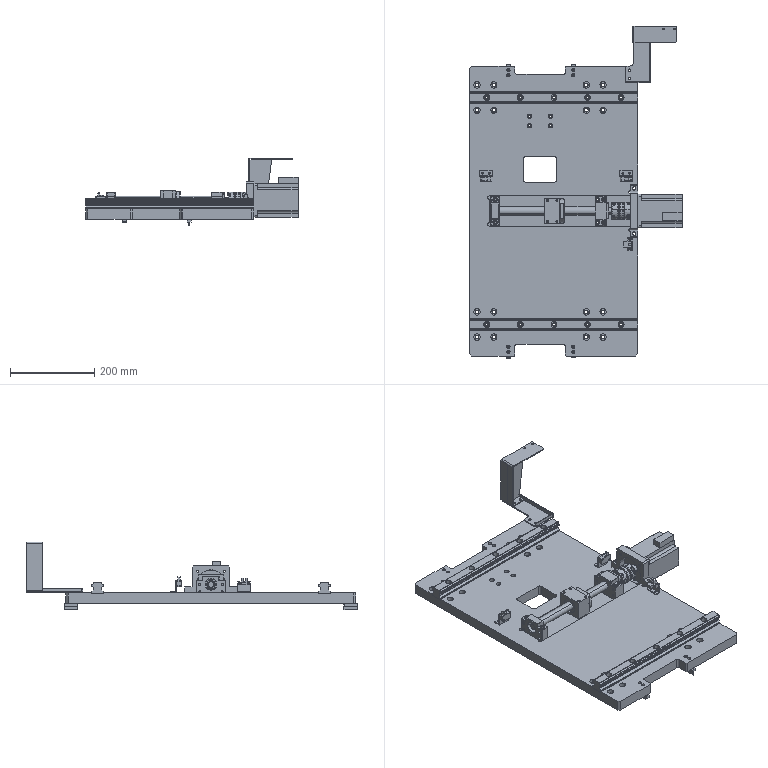Assembly | SolidWorks | mm | 27 component files | 28 solids | 1819 faces | box 505 x 789.7 x 161.7 mm | volume 7869612 mm3 | plane 909 | cylinder 651 | spline 127 | cone 126 | torus 6 | commonest cylinder face diameters 9 x52 5 x42 4 x40 15 x40 5.5 x40 6 x34 3.3 x32 4.2 x24
Bill of materials:
6G-DCSG-StopSwitchSeat | 2 |  | L-shaped angle bracket: a tall rectangular vertical plate joined at a right angle to a short horizontal foot. The vertical plate has four small holes near its upper portion and the foot has two larger holes.
6G-DCSG-ZeroPointSwitchSeat | 1 |  | L-shaped angle bracket: a wide rectangular vertical plate with a narrower horizontal foot. The vertical plate has two small holes near its top edge and the foot has two larger holes.
6G-HGR30-Y-Integrated | 2 |  | Long straight rail with a constant profile. Both sides have lengthwise grooves, and a row of evenly spaced counterbored holes runs along the top face.
6G-LimitSwitch | 2 |  | Small rectangular block with rounded corners and two through holes at diagonally opposite corners. On top there is a raised tab with a rounded end and a thin angled strip that slopes along the top face.
6G-OriginSwitch | 1 |  | Stepped rectangular block with two parallel upright prongs that form an open slot between them. Holes run both vertically and horizontally through the lower flange sections.
6G-TL06.01.02-XAxisMovingBasePlate | 1 |  | Large flat rectangular plate with many holes. It has a rectangular through-cutout, rectangular notches at both short ends, a shallow notch along one long edge, and shallow grooves or steps across the top face.
6G-TL06.01.05-DragChainFixingPlate | 1 |  | Formed thin-walled bracket: a tapered vertical web with a horizontal top flange and a horizontal bottom flange, joined by rounded bends. The top flange has two holes and the bottom flange has about three or four.
6G-TL06-StopBlock | 2 |  | Rectangular bar block with two round holes through its top face and one chamfered lower edge at one end.
6G-TL06-X-AxisCableCarrierBracket-A | 1 | AISI 304 | Thin flat plate with a stepped outline: a wide end and a narrower main body joined by a concave fillet. A narrow lip is turned down along one long edge. There are six round holes, and some corners are chamfered.
6G-TL06-X-AxisOrigin | 2 |  | Long bar with a T-shaped cross-section: a wide top flange over a narrower tongue underneath. Two round holes go into the top face.
6G-BF15SupportSide | 1 |  | Rectangular housing block with a raised centre section and a large central through bore. Four smaller holes go through the front face, two counterbored holes go down through the side shoulders, and the edges are chamfered.
6G-BK15FixedSide | 1 |  | Rectangular housing block with a raised centre section and a protruding flange boss on one face. A stepped central bore passes through it. There are four small holes around the bore on the boss, four through holes in the front face, and four counterbored vertical holes in the side shoulders.
6G-CPDW40-12-19 | 1 |  | Cylindrical body with a coaxial through-bore, made of two end hubs and a center ring. Thin disc-like layers sit in the gaps between them. Each hub has a slit and tangential cross holes with counterbores. The shape matches a clamp-style flexible shaft coupling.
6G-M4 | 4 |  | Headed fastener-like part: a cylindrical head with a hexagonal socket recess and a plain cylindrical shank with a chamfered tip. The shape matches a socket head cap screw.
6G-SGM7J-08A(750W) | 1 |  | Prismatic housing with a square front flange, four corner through-holes and a cylindrical output shaft sticking out from a round pilot boss. It has longitudinal grooves along the sides and a rectangular block on top. The shape matches a simplified motor (e.g., stepper or servo) envelope.
6G-TL06.01.03-X-AxisMotorMountingPlate | 1 |  | Flat rectangular plate with chamfered corners and a large central circular through-opening. Four small holes sit on a square pattern around the opening. Two side tabs at the base each have a through-hole perpendicular to the plate. The shape matches a mounting bracket or flange adapter plate.
6G-TL06.01.04-X-AxisFlangeMountingBlock | 1 |  | Rectangular block with a large circular through-bore along one axis. Four small holes surround the bore on the bore face, and four holes are in the top face. The shape matches a housing or nut block.
6G-TL06-Y-AxisFlange | 1 |  | Flanged cylindrical bushing with a central through-bore. The flange is round with two parallel flats and six through-holes. The shape matches a flanged lead-screw nut or flanged bushing.
6G-TL06-Y-AxisScrew | 1 |  | Long, slender stepped round shaft. A long main diameter steps down at one end into two progressively smaller journals. The other end has a short, slightly reduced section.
Mates:
1. concentric | 6G-DCSG-StopSwitchSeat-1 face at (-150.85, 83.8, 27) dir (0, 1, 0) r 1.25 | 6G-LimitSwitch-1 face at (-150.85, 71, 27) dir (0, 1, 0) r 1.75
2. coincident | 6G-DCSG-StopSwitchSeat-1 face at (-177, 83.8, 30) dir (0, 0, 1) | 6G-LimitSwitch-1 face at (-149.85, 81, 30) dir (0, 0, 1)
3. coincident | 6G-DCSG-StopSwitchSeat-1 face at (-177, 81, 30) dir (0, -1, 0) | 6G-LimitSwitch-1 face at (-149.85, 81, 16) dir (0, 1, 0)
4. concentric | 6G-DCSG-StopSwitchSeat-2 face at (160.85, 83.8, 27) dir (0, 1, 0) r 1.25 | 6G-LimitSwitch-2 face at (160.85, 81, 27) dir (0, -1, 0) r 1.75
5. coincident | 6G-DCSG-StopSwitchSeat-2 face at (157, 83.8, 30) dir (0, 0, 1) | 6G-LimitSwitch-2 face at (159.85, 71, 30) dir (0, 0, 1)
6. coincident | 6G-DCSG-StopSwitchSeat-2 face at (157, 81, 30) dir (0, -1, 0) | 6G-LimitSwitch-2 face at (159.85, 81, 16) dir (0, 1, 0)
7. concentric | 6G-DCSG-ZeroPointSwitchSeat-1 face at (184.472, -88.5, 22.3) dir (-1, 0, 0) r 1.25 | 6G-OriginSwitch-1 face at (187.872, -88.5, 22.3) dir (-1, 0, 0) r 1.5
8. parallel | 6G-DCSG-ZeroPointSwitchSeat-1 face at (187.272, -94, 26) dir (0, 0, 1) | 6G-OriginSwitch-1 face at (187.872, -95.044, 25.8) dir (0, 0, 1)
9. coincident | 6G-TL06.01.02-XAxisMovingBasePlate-1 face at (0, 0, -25) dir (0, 0, -1) | 6G-TL06-StopBlock-2 face at (-103.5, 349.7, -25) dir (0, 0, 1)
10. coincident | 6G-TL06.01.02-XAxisMovingBasePlate-1 face at (0, 0, -25) dir (0, 0, -1) | 6G-TL06-X-AxisOrigin-1 face at (46, 333, -25) dir (0, 0, 1)
11. coincident | 6G-TL06.01.02-XAxisMovingBasePlate-1 face at (0, 0, -25) dir (0, 0, -1) | 6G-TL06-StopBlock-2 face at (-103.5, 349.7, -25) dir (0, 0, 1)
12. coincident | 6G-TL06.01.02-XAxisMovingBasePlate-1 face at (0, 0, -25) dir (0, 0, -1) | 6G-TL06-X-AxisOrigin-1 face at (46, 333, -25) dir (0, 0, 1)
13. coincident | 6G-DCSG-StopSwitchSeat-1 face at (-177, 96, 0) dir (0, 0, -1) | 6G-TL06.01.02-XAxisMovingBasePlate-1 face at (0, 0, 0) dir (0, 0, 1)
14. coincident | 6G-DCSG-StopSwitchSeat-2 face at (157, 96, 0) dir (0, 0, -1) | 6G-TL06.01.02-XAxisMovingBasePlate-1 face at (0, 0, 0) dir (0, 0, 1)
15. coincident | 6G-DCSG-ZeroPointSwitchSeat-1 face at (175.272, -94, 0) dir (0, 0, -1) | 6G-TL06.01.02-XAxisMovingBasePlate-1 face at (0, 0, 0) dir (0, 0, 1)
16. coincident | 6G-TL06.01.02-XAxisMovingBasePlate-1 face at (0, 0, -2.5) dir (0, 0, 1) | 6G-HGR30-Y-Integrated-2 face at (-140, 262.25, -2.5) dir (0, 0, -1)
17. width | 6G-HGR30-Y-Integrated-2 face at (-140, 284, 2.61) dir (0, 1, 0) | 6G-HGR30-Y-Integrated-2 face at (-140, 256, -1) dir (0, -1, 0) | 6G-TL06.01.02-XAxisMovingBasePlate-1 face at (-200, 284, -2.5) dir (0, -1, 0) | 6G-TL06.01.02-XAxisMovingBasePlate-1 face at (-200, 256, -2.5) dir (0, 1, 0)
18. coincident | 6G-TL06.01.02-XAxisMovingBasePlate-1 face at (0, 0, -2.5) dir (0, 0, 1) | 6G-HGR30-Y-Integrated-3 face at (-140, -277.75, -2.5) dir (0, 0, -1)
19. width | 6G-HGR30-Y-Integrated-3 face at (-140, -284, -1) dir (0, -1, 0) | 6G-HGR30-Y-Integrated-3 face at (-140, -256, 2.61) dir (0, 1, 0) | 6G-TL06.01.02-XAxisMovingBasePlate-1 face at (-200, -284, -2.5) dir (0, 1, 0) | 6G-TL06.01.02-XAxisMovingBasePlate-1 face at (-200, -256, -2.5) dir (0, -1, 0)
20. width | 6G-HGR30-Y-Integrated-3 face at (-200, -220, -2.5) dir (-1, 0, 0) | 6G-HGR30-Y-Integrated-3 face at (200, -220, -2.5) dir (1, 0, 0) | 6G-TL06.01.02-XAxisMovingBasePlate-1 face at (200, -345, -25) dir (1, 0, 0) | 6G-TL06.01.02-XAxisMovingBasePlate-1 face at (-200, -345, -25) dir (-1, 0, 0)
21. width | 6G-HGR30-Y-Integrated-2 face at (-200, 320, -2.5) dir (-1, 0, 0) | 6G-HGR30-Y-Integrated-2 face at (200, 320, -2.5) dir (1, 0, 0) | 6G-TL06.01.02-XAxisMovingBasePlate-1 face at (200, -345, -25) dir (1, 0, 0) | 6G-TL06.01.02-XAxisMovingBasePlate-1 face at (-200, -345, -25) dir (-1, 0, 0)
22. coincident | 6G-TL06.01.02-XAxisMovingBasePlate-1 face at (0, 0, 0) dir (0, 0, 1) | 6G-TL06-Y-AxisMotorAssembly-2/6G-TL06.01.03-X-AxisMotorMountingPlate-1 face at (222.672, 45, 0) dir (0, 0, -1)
23. width | 6G-TL06-Y-AxisMotorAssembly-2/6G-TL06.01.03-X-AxisMotorMountingPlate-1 face at (222.672, 62, 0) dir (0, 1, 0) | 6G-TL06-Y-AxisMotorAssembly-2/6G-TL06.01.03-X-AxisMotorMountingPlate-1 face at (222.672, -62, 0) dir (0, -1, 0) | 6G-TL06.01.02-XAxisMovingBasePlate-1 face at (200, -45, -25) dir (0, 1, 0) | 6G-TL06.01.02-XAxisMovingBasePlate-1 face at (200, 45, -25) dir (0, -1, 0)
24. coincident | 6G-TL06.01.02-XAxisMovingBasePlate-1 face at (182, 45, -25) dir (1, 0, 0) | 6G-TL06-Y-AxisMotorAssembly-2/6G-TL06.01.03-X-AxisMotorMountingPlate-1 face at (182, 0, 21.75) dir (-1, 0, 0)
25. concentric | 6G-TL06.01.02-XAxisMovingBasePlate-1 face at (-108.5, 323, 0) dir (0, 0, 1) r 2.25 | 6G-TL06-StopBlock-2 face at (-108.5, 323, -25) dir (0, 0, 1) r 1.65
26. concentric | 6G-TL06.01.02-XAxisMovingBasePlate-1 face at (-108.5, 335, 0) dir (0, 0, 1) r 2.25 | 6G-TL06-StopBlock-2 face at (-108.5, 335, -25) dir (0, 0, 1) r 1.65
27. concentric | 6G-TL06.01.02-XAxisMovingBasePlate-1 face at (-108.5, -323, 0) dir (0, 0, 1) r 2.25 | 6G-TL06-StopBlock-3 face at (-108.5, -323, -25) dir (0, 0, 1) r 1.65
28. concentric | 6G-TL06.01.02-XAxisMovingBasePlate-1 face at (-108.5, -335, 0) dir (0, 0, 1) r 2.25 | 6G-TL06-StopBlock-3 face at (-108.5, -335, -25) dir (0, 0, 1) r 1.65
29. coincident | 6G-TL06.01.02-XAxisMovingBasePlate-1 face at (0, 0, -25) dir (0, 0, -1) | 6G-TL06-StopBlock-3 face at (-113.5, -349.7, -25) dir (0, 0, 1)
30. concentric | 6G-TL06.01.02-XAxisMovingBasePlate-1 face at (46, 323, 0) dir (0, 0, 1) r 2.25 | 6G-TL06-X-AxisOrigin-1 face at (46, 323, -31.5) dir (0, 0, -1) r 1.65
31. concentric | 6G-TL06.01.02-XAxisMovingBasePlate-1 face at (46, 335, 0) dir (0, 0, 1) r 2.25 | 6G-TL06-X-AxisOrigin-1 face at (46, 335, -31.5) dir (0, 0, -1) r 1.65
32. concentric | 6G-DCSG-StopSwitchSeat-2 face at (164, 90, -7.2) dir (0, 0, 1) r 2.1 | 6G-TL06.01.02-XAxisMovingBasePlate-1 face at (164, 90, 0) dir (0, 0, 1) r 1.65
33. concentric | 6G-DCSG-StopSwitchSeat-2 face at (180, 90, -7.2) dir (0, 0, 1) r 2.1 | 6G-TL06.01.02-XAxisMovingBasePlate-1 face at (180, 90, 0) dir (0, 0, 1) r 1.65
34. concentric | 6G-DCSG-ZeroPointSwitchSeat-1 face at (180, -72, -27.2) dir (0, 0, 1) r 2.1 | 6G-TL06.01.02-XAxisMovingBasePlate-1 face at (180, -72, 0) dir (0, 0, 1) r 1.65
35. concentric | 6G-DCSG-ZeroPointSwitchSeat-1 face at (180, -86, -27.2) dir (0, 0, 1) r 2.1 | 6G-TL06.01.02-XAxisMovingBasePlate-1 face at (180, -86, 0) dir (0, 0, 1) r 1.65
36. concentric | 6G-DCSG-StopSwitchSeat-1 face at (-170, 90, -7.2) dir (0, 0, 1) r 2.1 | 6G-TL06.01.02-XAxisMovingBasePlate-1 face at (-170, 90, 0) dir (0, 0, 1) r 1.65
37. concentric | 6G-DCSG-StopSwitchSeat-1 face at (-154, 90, -7.2) dir (0, 0, 1) r 2.1 | 6G-TL06.01.02-XAxisMovingBasePlate-1 face at (-154, 90, 0) dir (0, 0, 1) r 1.65
38. coincident | 6G-TL06.01.02-XAxisMovingBasePlate-1 face at (0, 0, 0) dir (0, 0, 1) | 6G-TL06-X-AxisCableCarrierBracket-A-1 face at (180, 355, 0) dir (0, 0, -1)
39. concentric | 6G-TL06.01.02-XAxisMovingBasePlate-1 face at (180, 315, 0) dir (0, 0, 1) r 2.5 | 6G-TL06-X-AxisCableCarrierBracket-A-1 face at (180, 315, 0) dir (0, 0, 1) r 3.1
40. concentric | 6G-TL06.01.02-XAxisMovingBasePlate-1 face at (180, 335, 0) dir (0, 0, 1) r 2.5 | 6G-TL06-X-AxisCableCarrierBracket-A-1 face at (180, 335, 0) dir (0, 0, 1) r 3.1
41. coincident | 6G-TL06.01.05-DragChainFixingPlate-1 face at (207.375, 411.5, 2.5) dir (0, 0, -1) | 6G-TL06-X-AxisCableCarrierBracket-A-1 face at (180, 355, 2.5) dir (0, 0, 1)
42. coincident | 6G-TL06.01.05-DragChainFixingPlate-1 face at (187.25, 440, 2.5) dir (0, 1, 0) | 6G-TL06-X-AxisCableCarrierBracket-A-1 edge at (227, 440, 0) dir (-1, 0, 0)
43. coincident | 6G-TL06.01.05-DragChainFixingPlate-1 face at (227.5, 440, 2.5) dir (1, 0, 0) | 6G-TL06-X-AxisCableCarrierBracket-A-1 face at (227.5, 305, 2.5) dir (-1, 0, 0)
44. coincident | 6G-DCSG-ZeroPointSwitchSeat-1 face at (184.472, -94, 30) dir (-1, 0, 0) | 6G-OriginSwitch-1 face at (184.472, -92.25, 15.8) dir (1, 0, 0)
45. concentric | 6G-TL06.01.02-XAxisMovingBasePlate-1 face at (46, -323, 0) dir (0, 0, 1) r 4 | 6G-TL06-X-AxisOrigin-2 face at (46, -323, -31.5) dir (0, 0, -1) r 1.65
46. concentric | 6G-TL06.01.02-XAxisMovingBasePlate-1 face at (46, -335, 0) dir (0, 0, 1) r 4 | 6G-TL06-X-AxisOrigin-2 face at (46, -335, -31.5) dir (0, 0, -1) r 1.65
47. coincident | 6G-TL06.01.02-XAxisMovingBasePlate-1 face at (0, 0, -25) dir (0, 0, -1) | 6G-TL06-X-AxisOrigin-2 face at (46, -333, -25) dir (0, 0, 1)
48. concentric | 6G-TL06-Y-AxisScrew-1 face at (-1.75, 0, 84) dir (0, 0, 1) r 10 | 6G-BK15FixedSide-1 face at (-1.75, 0, 57) dir (0, 0, 1) r 7.5
49. coincident | 6G-TL06-Y-AxisScrew-1 face at (-1.75, 0, 84) dir (0, 0, -1) | 6G-BK15FixedSide-1 face at (-29.75, 0, 84) dir (0, 0, 1)
50. parallel | 6G-BK15FixedSide-1 face at (18.25, 20, 57) dir (1, 0, 0) | 6G-BF15SupportSide-1 face at (18.25, 19, 312) dir (1, 0, 0)
51. concentric | 6G-TL06-Y-AxisScrew-1 face at (-1.75, 0, 84) dir (0, 0, 1) r 10 | 6G-BF15SupportSide-1 face at (-1.75, 0, 312) dir (0, 0, 1) r 13
52. distance | 6G-BF15SupportSide-1 face at (-29.75, 0, 312) dir (0, 0, -1) | 6G-BK15FixedSide-1 face at (-29.75, 0, 84) dir (0, 0, 1)
53. concentric | 6G-TL06-Y-AxisScrew-1 face at (-1.75, 0, 24) dir (0, 0, 1) r 6 | 6G-TL06.01.03-X-AxisMotorMountingPlate-1 face at (-1.75, 0, -18) dir (0, 0, 1) r 35
54. parallel | 6G-BK15FixedSide-1 face at (18.25, 20, 57) dir (1, 0, 0) | 6G-TL06.01.03-X-AxisMotorMountingPlate-1 face at (42.25, -60, -18) dir (1, 0, 0)
55. coordinate | 6G-TL06.01.03-X-AxisMotorMountingPlate-1 sketch point at (0, 0, 0) dir (1, 0, 0) | 6G-TL06-Y-AxisMotorAssembly sketch point at (0, 0, 0) dir (1, 0, 0)
56. concentric | 6G-TL06.01.03-X-AxisMotorMountingPlate-1 face at (-1.75, 0, -18) dir (0, 0, 1) r 35 | 6G-SGM7J-08A(750W)-1 face at (-1.75, 0, 22) dir (0, 0, -1) r 9.5
57. concentric | 6G-TL06.01.03-X-AxisMotorMountingPlate-1 face at (30.07, 31.82, 0) dir (0, 0, 1) r 2.5 | 6G-SGM7J-08A(750W)-1 face at (30.07, 31.82, -26) dir (0, 0, 1) r 3.5
58. coincident | 6G-TL06.01.03-X-AxisMotorMountingPlate-1 face at (0, 0, -18) dir (0, 0, -1) | 6G-SGM7J-08A(750W)-1 face at (-36.913, -35.163, -18) dir (0, 0, 1)
59. distance | 6G-TL06-Y-AxisScrew-1 face at (-1.75, 0, 24) dir (0, 0, -1) | 6G-SGM7J-08A(750W)-1 face at (-1.75, 0, 22) dir (0, 0, 1)
60. concentric | 6G-TL06-Y-AxisScrew-1 face at (-1.75, 0, 84) dir (0, 0, 1) r 10 | 6G-TL06-Y-AxisFlange-1 face at (-1.75, 0, 201.964) dir (0, 0, -1) r 18
61. parallel | 6G-BK15FixedSide-1 face at (18.25, 20, 57) dir (1, 0, 0) | 6G-TL06-Y-AxisFlange-1 face at (20.25, 25.545, 201.964) dir (1, 0, 0)
62. concentric | 6G-TL06.01.04-X-AxisFlangeMountingBlock-1 face at (-1.75, 0, 203.964) dir (0, 0, -1) r 18.25 | 6G-TL06-Y-AxisFlange-1 face at (-1.75, 0, 201.964) dir (0, 0, -1) r 18
63. concentric | 6G-TL06.01.04-X-AxisFlangeMountingBlock-1 face at (14.867, 16.617, 167.964) dir (0, 0, -1) r 2.1 | 6G-TL06-Y-AxisFlange-1 face at (14.867, 16.617, 201.964) dir (0, 0, -1) r 3.3
64. coincident | 6G-TL06.01.04-X-AxisFlangeMountingBlock-1 face at (20.95, -30, 167.964) dir (0, 0, -1) | 6G-TL06-Y-AxisFlange-1 face at (-1.75, 0, 167.964) dir (0, 0, 1)
65. concentric | 6G-SGM7J-08A(750W)-1 face at (-1.75, 0, 22) dir (0, 0, -1) r 9.5 | 6G-CPDW40-12-19-1/6G-CPDW40-12-19.stp-1/6G-CPDW40-12-19-1 face at (-1.75, 0, 0) dir (0, 0, 1) r 20
66. coincident | 6G-TL06-Y-AxisScrew-1 face at (-1.75, 0, 44) dir (0, 0, -1) | 6G-CPDW40-12-19-1/6G-CPDW40-12-19.stp-1/6G-CPDW40-12-19-1 face at (-4.472, 19.309, 44) dir (0, 0, 1)